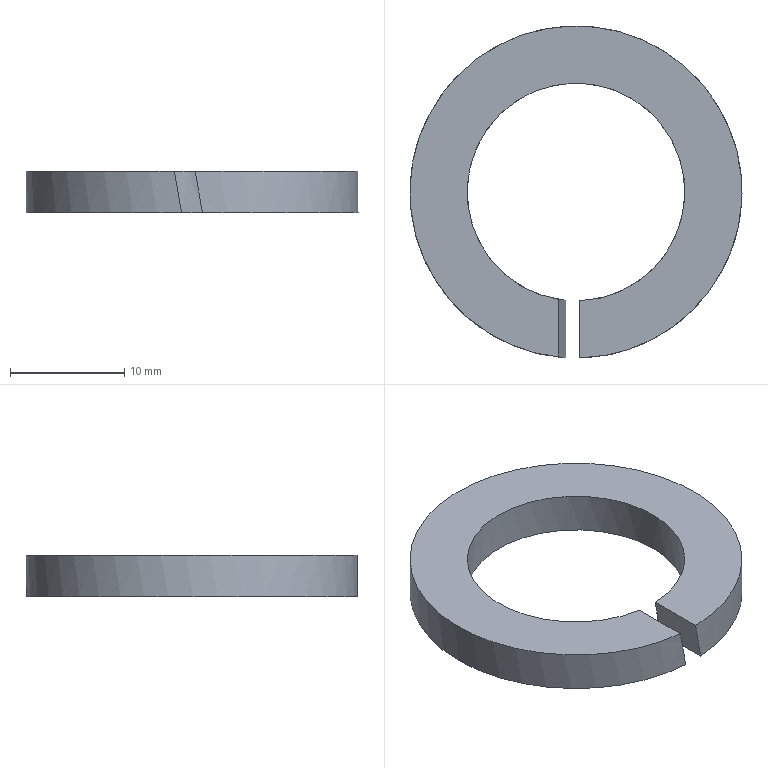Component | NX | GB859-87__18 | 1 solid | 6 faces | box 29.04 x 29.04 x 3.6 mm | volume 1326 mm3 | plane 4 | cylinder 2 | commonest cylinder face diameters 29.04 x1 19.04 x1
STEP:
#1=CARTESIAN_POINT('',(0.,0.,0.));
#2=DIRECTION('',(0.,0.,1.));
#3=DIRECTION('',(1.,0.,0.));
#4=AXIS2_PLACEMENT_3D('',#1,#2,#3);
#5=CARTESIAN_POINT('',(-0.9152,-14.493,110.));
#6=VERTEX_POINT('',#5);
#7=CARTESIAN_POINT('',(0.9125,-14.493,110.));
#8=VERTEX_POINT('',#7);
#9=CARTESIAN_POINT('',(-0.001341,-0.001341,110.));
#10=DIRECTION('',(0.,0.,-1.));
#11=DIRECTION('',(0.,1.,0.));
#12=AXIS2_PLACEMENT_3D('',#9,#10,#11);
#13=CIRCLE('',#12,14.52);
#14=CARTESIAN_POINT('',(-0.001341,-0.001341,110.));
#15=DIRECTION('',(0.,0.,-1.));
#16=DIRECTION('',(0.,1.,0.));
#17=AXIS2_PLACEMENT_3D('',#14,#15,#16);
#18=CYLINDRICAL_SURFACE('',#17,14.52);
#19=CARTESIAN_POINT('',(-6.283,0.));
#20=DIRECTION('',(1.,0.));
#21=VECTOR('',#20,1.);
#22=LINE('',#19,#21);
#23=(GEOMETRIC_REPRESENTATION_CONTEXT(2)PARAMETRIC_REPRESENTATION_CONTEXT()REPRESENTATION_CONTEXT('',''));
#24=DEFINITIONAL_REPRESENTATION('',(#22),#23);
#25=PCURVE('',#18,#24);
#26=CARTESIAN_POINT('',(9.519,-0.001341,110.));
#27=DIRECTION('',(0.,0.,-1.));
#28=DIRECTION('',(0.,1.,0.));
#29=AXIS2_PLACEMENT_3D('',#26,#27,#28);
#30=PLANE('',#29);
#31=CARTESIAN_POINT('',(0.,-9.52));
#32=DIRECTION('',(1.,0.));
#33=AXIS2_PLACEMENT_2D('',#31,#32);
#34=CIRCLE('',#33,14.52);
#35=(GEOMETRIC_REPRESENTATION_CONTEXT(2)PARAMETRIC_REPRESENTATION_CONTEXT()REPRESENTATION_CONTEXT('',''));
#36=DEFINITIONAL_REPRESENTATION('',(#34),#35);
#37=PCURVE('',#30,#36);
#38=SURFACE_CURVE('',#13,(#25,#37),.PCURVE_S1.);
#39=EDGE_CURVE('',#6,#8,#38,.T.);
#40=ORIENTED_EDGE('',*,*,#39,.F.);
#41=CARTESIAN_POINT('',(-1.55,-14.439,113.6));
#42=VERTEX_POINT('',#41);
#43=CARTESIAN_POINT('',(-0.001341,-0.001341,104.817));
#44=DIRECTION('',(-0.9848,0.,-0.1736));
#45=DIRECTION('',(0.1736,0.,-0.9848));
#46=AXIS2_PLACEMENT_3D('',#43,#44,#45);
#47=ELLIPSE('',#46,83.617,14.52);
#48=CARTESIAN_POINT('',(-3.079,-0.));
#49=CARTESIAN_POINT('',(-3.035,-3.6));
#50=B_SPLINE_CURVE_WITH_KNOTS('',1,(#48,#49),.UNSPECIFIED.,.F.,.F.,(2,2),(1.634,1.678),.PIECEWISE_BEZIER_KNOTS.);
#51=(GEOMETRIC_REPRESENTATION_CONTEXT(2)PARAMETRIC_REPRESENTATION_CONTEXT()REPRESENTATION_CONTEXT('',''));
#52=DEFINITIONAL_REPRESENTATION('',(#50),#51);
#53=PCURVE('',#18,#52);
#54=CARTESIAN_POINT('',(-2.19,-21.781,117.23));
#55=DIRECTION('',(0.9848,0.,0.1736));
#56=DIRECTION('',(-0.1736,0.,0.9848));
#57=AXIS2_PLACEMENT_3D('',#54,#55,#56);
#58=PLANE('',#57);
#59=CARTESIAN_POINT('',(-96.222,-21.78));
#60=CARTESIAN_POINT('',(-96.222,3.369));
#61=CARTESIAN_POINT('',(29.205,-9.205));
#62=CARTESIAN_POINT('',(154.631,-21.78));
#63=CARTESIAN_POINT('',(29.205,-34.355));
#64=CARTESIAN_POINT('',(-96.222,-46.929));
#65=CARTESIAN_POINT('',(-96.222,-21.78));
#66=(BOUNDED_CURVE()B_SPLINE_CURVE(2,(#59,#60,#61,#62,#63,#64,#65),.UNSPECIFIED.,.T.,.F.)B_SPLINE_CURVE_WITH_KNOTS((1,2,2,2,2,1),(-2.094,0.,2.094,4.189,6.283,8.378),.UNSPECIFIED.)CURVE()GEOMETRIC_REPRESENTATION_ITEM()RATIONAL_B_SPLINE_CURVE((1.,0.5,1.,0.5,1.,0.5,1.))REPRESENTATION_ITEM(''));
#67=(GEOMETRIC_REPRESENTATION_CONTEXT(2)PARAMETRIC_REPRESENTATION_CONTEXT()REPRESENTATION_CONTEXT('',''));
#68=DEFINITIONAL_REPRESENTATION('',(#66),#67);
#69=PCURVE('',#58,#68);
#70=SURFACE_CURVE('',#47,(#53,#69),.PCURVE_S1.);
#71=EDGE_CURVE('',#6,#42,#70,.T.);
#72=ORIENTED_EDGE('',*,*,#71,.T.);
#73=CARTESIAN_POINT('',(0.2778,-14.519,113.6));
#74=VERTEX_POINT('',#73);
#75=CARTESIAN_POINT('',(-0.001341,-0.001341,113.6));
#76=DIRECTION('',(0.,0.,-1.));
#77=DIRECTION('',(0.,1.,0.));
#78=AXIS2_PLACEMENT_3D('',#75,#76,#77);
#79=CIRCLE('',#78,14.52);
#80=CARTESIAN_POINT('',(-6.283,-3.6));
#81=DIRECTION('',(1.,0.));
#82=VECTOR('',#81,1.);
#83=LINE('',#80,#82);
#84=(GEOMETRIC_REPRESENTATION_CONTEXT(2)PARAMETRIC_REPRESENTATION_CONTEXT()REPRESENTATION_CONTEXT('',''));
#85=DEFINITIONAL_REPRESENTATION('',(#83),#84);
#86=PCURVE('',#18,#85);
#87=CARTESIAN_POINT('',(14.519,-0.001341,113.6));
#88=DIRECTION('',(0.,0.,1.));
#89=DIRECTION('',(0.,-1.,0.));
#90=AXIS2_PLACEMENT_3D('',#87,#88,#89);
#91=PLANE('',#90);
#92=CARTESIAN_POINT('',(-14.52,-14.52));
#93=CARTESIAN_POINT('',(-14.52,10.629));
#94=CARTESIAN_POINT('',(7.26,-1.945));
#95=CARTESIAN_POINT('',(29.04,-14.52));
#96=CARTESIAN_POINT('',(7.26,-27.095));
#97=CARTESIAN_POINT('',(-14.52,-39.669));
#98=CARTESIAN_POINT('',(-14.52,-14.52));
#99=(BOUNDED_CURVE()B_SPLINE_CURVE(2,(#92,#93,#94,#95,#96,#97,#98),.UNSPECIFIED.,.T.,.F.)B_SPLINE_CURVE_WITH_KNOTS((1,2,2,2,2,1),(-2.094,0.,2.094,4.189,6.283,8.378),.UNSPECIFIED.)CURVE()GEOMETRIC_REPRESENTATION_ITEM()RATIONAL_B_SPLINE_CURVE((1.,0.5,1.,0.5,1.,0.5,1.))REPRESENTATION_ITEM(''));
#100=(GEOMETRIC_REPRESENTATION_CONTEXT(2)PARAMETRIC_REPRESENTATION_CONTEXT()REPRESENTATION_CONTEXT('',''));
#101=DEFINITIONAL_REPRESENTATION('',(#99),#100);
#102=PCURVE('',#91,#101);
#103=SURFACE_CURVE('',#79,(#86,#102),.PCURVE_S1.);
#104=EDGE_CURVE('',#42,#74,#103,.T.);
#105=ORIENTED_EDGE('',*,*,#104,.T.);
#106=CARTESIAN_POINT('',(-0.001341,-0.001341,115.183));
#107=DIRECTION('',(0.9848,0.,0.1736));
#108=DIRECTION('',(0.1736,0.,-0.9848));
#109=AXIS2_PLACEMENT_3D('',#106,#107,#108);
#110=ELLIPSE('',#109,83.617,14.52);
#111=CARTESIAN_POINT('',(3.122,-3.6));
#112=CARTESIAN_POINT('',(3.079,0.));
#113=B_SPLINE_CURVE_WITH_KNOTS('',1,(#111,#112),.UNSPECIFIED.,.F.,.F.,(2,2),(4.732,4.775),.PIECEWISE_BEZIER_KNOTS.);
#114=(GEOMETRIC_REPRESENTATION_CONTEXT(2)PARAMETRIC_REPRESENTATION_CONTEXT()REPRESENTATION_CONTEXT('',''));
#115=DEFINITIONAL_REPRESENTATION('',(#113),#114);
#116=PCURVE('',#18,#115);
#117=CARTESIAN_POINT('',(2.187,-21.781,102.77));
#118=DIRECTION('',(-0.9848,0.,-0.1736));
#119=DIRECTION('',(0.1736,0.,-0.9848));
#120=AXIS2_PLACEMENT_3D('',#117,#118,#119);
#121=PLANE('',#120);
#122=CARTESIAN_POINT('',(71.013,-21.78));
#123=CARTESIAN_POINT('',(71.013,-46.929));
#124=CARTESIAN_POINT('',(-54.413,-34.355));
#125=CARTESIAN_POINT('',(-179.839,-21.78));
#126=CARTESIAN_POINT('',(-54.413,-9.205));
#127=CARTESIAN_POINT('',(71.013,3.369));
#128=CARTESIAN_POINT('',(71.013,-21.78));
#129=(BOUNDED_CURVE()B_SPLINE_CURVE(2,(#122,#123,#124,#125,#126,#127,#128),.UNSPECIFIED.,.T.,.F.)B_SPLINE_CURVE_WITH_KNOTS((1,2,2,2,2,1),(-2.094,0.,2.094,4.189,6.283,8.378),.UNSPECIFIED.)CURVE()GEOMETRIC_REPRESENTATION_ITEM()RATIONAL_B_SPLINE_CURVE((1.,0.5,1.,0.5,1.,0.5,1.))REPRESENTATION_ITEM(''));
#130=(GEOMETRIC_REPRESENTATION_CONTEXT(2)PARAMETRIC_REPRESENTATION_CONTEXT()REPRESENTATION_CONTEXT('',''));
#131=DEFINITIONAL_REPRESENTATION('',(#129),#130);
#132=PCURVE('',#121,#131);
#133=SURFACE_CURVE('',#110,(#116,#132),.PCURVE_S1.);
#134=EDGE_CURVE('',#74,#8,#133,.T.);
#135=ORIENTED_EDGE('',*,*,#134,.T.);
#136=EDGE_LOOP('',(#40,#72,#105,#135));
#137=FACE_BOUND('',#136,.T.);
#138=ADVANCED_FACE('',(#137),#18,.T.);
#139=ORIENTED_EDGE('',*,*,#104,.F.);
#140=CARTESIAN_POINT('',(-1.55,-9.395,113.6));
#141=VERTEX_POINT('',#140);
#142=CARTESIAN_POINT('',(-1.55,-0.001341,113.6));
#143=DIRECTION('',(0.,1.,0.));
#144=VECTOR('',#143,1.);
#145=LINE('',#142,#144);
#146=CARTESIAN_POINT('',(0.,-16.069));
#147=DIRECTION('',(-1.,0.));
#148=VECTOR('',#147,1.);
#149=LINE('',#146,#148);
#150=(GEOMETRIC_REPRESENTATION_CONTEXT(2)PARAMETRIC_REPRESENTATION_CONTEXT()REPRESENTATION_CONTEXT('',''));
#151=DEFINITIONAL_REPRESENTATION('',(#149),#150);
#152=PCURVE('',#91,#151);
#153=CARTESIAN_POINT('',(-3.686,-21.78));
#154=DIRECTION('',(0.,-1.));
#155=VECTOR('',#154,1.);
#156=LINE('',#153,#155);
#157=(GEOMETRIC_REPRESENTATION_CONTEXT(2)PARAMETRIC_REPRESENTATION_CONTEXT()REPRESENTATION_CONTEXT('',''));
#158=DEFINITIONAL_REPRESENTATION('',(#156),#157);
#159=PCURVE('',#58,#158);
#160=SURFACE_CURVE('',#145,(#152,#159),.PCURVE_S1.);
#161=EDGE_CURVE('',#42,#141,#160,.T.);
#162=ORIENTED_EDGE('',*,*,#161,.T.);
#163=CARTESIAN_POINT('',(0.2778,-9.517,113.6));
#164=VERTEX_POINT('',#163);
#165=CARTESIAN_POINT('',(-0.001341,-0.001341,113.6));
#166=DIRECTION('',(0.,0.,-1.));
#167=DIRECTION('',(0.,1.,0.));
#168=AXIS2_PLACEMENT_3D('',#165,#166,#167);
#169=CIRCLE('',#168,9.52);
#170=CARTESIAN_POINT('',(-9.52,-14.52));
#171=CARTESIAN_POINT('',(-9.52,1.969));
#172=CARTESIAN_POINT('',(4.76,-6.275));
#173=CARTESIAN_POINT('',(19.04,-14.52));
#174=CARTESIAN_POINT('',(4.76,-22.765));
#175=CARTESIAN_POINT('',(-9.52,-31.009));
#176=CARTESIAN_POINT('',(-9.52,-14.52));
#177=(BOUNDED_CURVE()B_SPLINE_CURVE(2,(#170,#171,#172,#173,#174,#175,#176),.UNSPECIFIED.,.T.,.F.)B_SPLINE_CURVE_WITH_KNOTS((1,2,2,2,2,1),(-2.094,0.,2.094,4.189,6.283,8.378),.UNSPECIFIED.)CURVE()GEOMETRIC_REPRESENTATION_ITEM()RATIONAL_B_SPLINE_CURVE((1.,0.5,1.,0.5,1.,0.5,1.))REPRESENTATION_ITEM(''));
#178=(GEOMETRIC_REPRESENTATION_CONTEXT(2)PARAMETRIC_REPRESENTATION_CONTEXT()REPRESENTATION_CONTEXT('',''));
#179=DEFINITIONAL_REPRESENTATION('',(#177),#178);
#180=PCURVE('',#91,#179);
#181=CARTESIAN_POINT('',(-0.001341,-0.001341,110.));
#182=DIRECTION('',(0.,0.,-1.));
#183=DIRECTION('',(0.,1.,0.));
#184=AXIS2_PLACEMENT_3D('',#181,#182,#183);
#185=CYLINDRICAL_SURFACE('',#184,9.52);
#186=CARTESIAN_POINT('',(-6.283,-3.6));
#187=DIRECTION('',(1.,0.));
#188=VECTOR('',#187,1.);
#189=LINE('',#186,#188);
#190=(GEOMETRIC_REPRESENTATION_CONTEXT(2)PARAMETRIC_REPRESENTATION_CONTEXT()REPRESENTATION_CONTEXT('',''));
#191=DEFINITIONAL_REPRESENTATION('',(#189),#190);
#192=PCURVE('',#185,#191);
#193=SURFACE_CURVE('',#169,(#180,#192),.PCURVE_S1.);
#194=EDGE_CURVE('',#141,#164,#193,.T.);
#195=ORIENTED_EDGE('',*,*,#194,.T.);
#196=CARTESIAN_POINT('',(0.2778,-0.001341,113.6));
#197=DIRECTION('',(0.,-1.,0.));
#198=VECTOR('',#197,1.);
#199=LINE('',#196,#198);
#200=CARTESIAN_POINT('',(0.,-14.241));
#201=DIRECTION('',(1.,0.));
#202=VECTOR('',#201,1.);
#203=LINE('',#200,#202);
#204=(GEOMETRIC_REPRESENTATION_CONTEXT(2)PARAMETRIC_REPRESENTATION_CONTEXT()REPRESENTATION_CONTEXT('',''));
#205=DEFINITIONAL_REPRESENTATION('',(#203),#204);
#206=PCURVE('',#91,#205);
#207=CARTESIAN_POINT('',(-10.997,-21.78));
#208=DIRECTION('',(0.,1.));
#209=VECTOR('',#208,1.);
#210=LINE('',#207,#209);
#211=(GEOMETRIC_REPRESENTATION_CONTEXT(2)PARAMETRIC_REPRESENTATION_CONTEXT()REPRESENTATION_CONTEXT('',''));
#212=DEFINITIONAL_REPRESENTATION('',(#210),#211);
#213=PCURVE('',#121,#212);
#214=SURFACE_CURVE('',#199,(#206,#213),.PCURVE_S1.);
#215=EDGE_CURVE('',#164,#74,#214,.T.);
#216=ORIENTED_EDGE('',*,*,#215,.T.);
#217=EDGE_LOOP('',(#139,#162,#195,#216));
#218=FACE_BOUND('',#217,.T.);
#219=ADVANCED_FACE('',(#218),#91,.T.);
#220=CARTESIAN_POINT('',(0.9125,-9.477,110.));
#221=VERTEX_POINT('',#220);
#222=CARTESIAN_POINT('',(-0.001341,-0.001341,115.183));
#223=DIRECTION('',(-0.9848,0.,-0.1736));
#224=DIRECTION('',(0.1736,0.,-0.9848));
#225=AXIS2_PLACEMENT_3D('',#222,#223,#224);
#226=ELLIPSE('',#225,54.823,9.52);
#227=CARTESIAN_POINT('',(3.045,0.));
#228=CARTESIAN_POINT('',(3.112,-3.6));
#229=B_SPLINE_CURVE_WITH_KNOTS('',1,(#227,#228),.UNSPECIFIED.,.F.,.F.,(2,2),(1.475,1.541),.PIECEWISE_BEZIER_KNOTS.);
#230=(GEOMETRIC_REPRESENTATION_CONTEXT(2)PARAMETRIC_REPRESENTATION_CONTEXT()REPRESENTATION_CONTEXT('',''));
#231=DEFINITIONAL_REPRESENTATION('',(#229),#230);
#232=PCURVE('',#185,#231);
#233=CARTESIAN_POINT('',(-12.604,-21.78));
#234=DIRECTION('',(1.,0.));
#235=AXIS2_PLACEMENT_2D('',#233,#234);
#236=ELLIPSE('',#235,54.823,9.52);
#237=(GEOMETRIC_REPRESENTATION_CONTEXT(2)PARAMETRIC_REPRESENTATION_CONTEXT()REPRESENTATION_CONTEXT('',''));
#238=DEFINITIONAL_REPRESENTATION('',(#236),#237);
#239=PCURVE('',#121,#238);
#240=SURFACE_CURVE('',#226,(#232,#239),.PCURVE_S1.);
#241=EDGE_CURVE('',#221,#164,#240,.T.);
#242=ORIENTED_EDGE('',*,*,#241,.F.);
#243=CARTESIAN_POINT('',(-0.9152,-9.477,110.));
#244=VERTEX_POINT('',#243);
#245=CARTESIAN_POINT('',(-0.001341,-0.001341,110.));
#246=DIRECTION('',(0.,0.,-1.));
#247=DIRECTION('',(0.,1.,0.));
#248=AXIS2_PLACEMENT_3D('',#245,#246,#247);
#249=CIRCLE('',#248,9.52);
#250=CARTESIAN_POINT('',(-6.283,0.));
#251=DIRECTION('',(1.,0.));
#252=VECTOR('',#251,1.);
#253=LINE('',#250,#252);
#254=(GEOMETRIC_REPRESENTATION_CONTEXT(2)PARAMETRIC_REPRESENTATION_CONTEXT()REPRESENTATION_CONTEXT('',''));
#255=DEFINITIONAL_REPRESENTATION('',(#253),#254);
#256=PCURVE('',#185,#255);
#257=CARTESIAN_POINT('',(0.,-9.52));
#258=DIRECTION('',(1.,0.));
#259=AXIS2_PLACEMENT_2D('',#257,#258);
#260=CIRCLE('',#259,9.52);
#261=(GEOMETRIC_REPRESENTATION_CONTEXT(2)PARAMETRIC_REPRESENTATION_CONTEXT()REPRESENTATION_CONTEXT('',''));
#262=DEFINITIONAL_REPRESENTATION('',(#260),#261);
#263=PCURVE('',#30,#262);
#264=SURFACE_CURVE('',#249,(#256,#263),.PCURVE_S1.);
#265=EDGE_CURVE('',#244,#221,#264,.T.);
#266=ORIENTED_EDGE('',*,*,#265,.F.);
#267=CARTESIAN_POINT('',(-0.001341,-0.001341,104.817));
#268=DIRECTION('',(0.9848,0.,0.1736));
#269=DIRECTION('',(0.1736,0.,-0.9848));
#270=AXIS2_PLACEMENT_3D('',#267,#268,#269);
#271=ELLIPSE('',#270,54.823,9.52);
#272=CARTESIAN_POINT('',(-2.978,-3.6));
#273=CARTESIAN_POINT('',(-3.045,0.));
#274=B_SPLINE_CURVE_WITH_KNOTS('',1,(#272,#273),.UNSPECIFIED.,.F.,.F.,(2,2),(4.549,4.616),.PIECEWISE_BEZIER_KNOTS.);
#275=(GEOMETRIC_REPRESENTATION_CONTEXT(2)PARAMETRIC_REPRESENTATION_CONTEXT()REPRESENTATION_CONTEXT('',''));
#276=DEFINITIONAL_REPRESENTATION('',(#274),#275);
#277=PCURVE('',#185,#276);
#278=CARTESIAN_POINT('',(-12.604,-21.78));
#279=DIRECTION('',(-1.,0.));
#280=AXIS2_PLACEMENT_2D('',#278,#279);
#281=ELLIPSE('',#280,54.823,9.52);
#282=(GEOMETRIC_REPRESENTATION_CONTEXT(2)PARAMETRIC_REPRESENTATION_CONTEXT()REPRESENTATION_CONTEXT('',''));
#283=DEFINITIONAL_REPRESENTATION('',(#281),#282);
#284=PCURVE('',#58,#283);
#285=SURFACE_CURVE('',#271,(#277,#284),.PCURVE_S1.);
#286=EDGE_CURVE('',#141,#244,#285,.T.);
#287=ORIENTED_EDGE('',*,*,#286,.F.);
#288=ORIENTED_EDGE('',*,*,#194,.T.);
#289=EDGE_LOOP('',(#242,#266,#287,#288));
#290=FACE_BOUND('',#289,.F.);
#291=ADVANCED_FACE('',(#290),#185,.F.);
#292=ORIENTED_EDGE('',*,*,#265,.F.);
#293=CARTESIAN_POINT('',(-0.9152,-0.001341,110.));
#294=DIRECTION('',(0.,-1.,0.));
#295=VECTOR('',#294,1.);
#296=LINE('',#293,#295);
#297=CARTESIAN_POINT('',(0.,-10.434));
#298=DIRECTION('',(-1.,0.));
#299=VECTOR('',#298,1.);
#300=LINE('',#297,#299);
#301=(GEOMETRIC_REPRESENTATION_CONTEXT(2)PARAMETRIC_REPRESENTATION_CONTEXT()REPRESENTATION_CONTEXT('',''));
#302=DEFINITIONAL_REPRESENTATION('',(#300),#301);
#303=PCURVE('',#30,#302);
#304=CARTESIAN_POINT('',(-7.341,-21.78));
#305=DIRECTION('',(0.,1.));
#306=VECTOR('',#305,1.);
#307=LINE('',#304,#306);
#308=(GEOMETRIC_REPRESENTATION_CONTEXT(2)PARAMETRIC_REPRESENTATION_CONTEXT()REPRESENTATION_CONTEXT('',''));
#309=DEFINITIONAL_REPRESENTATION('',(#307),#308);
#310=PCURVE('',#58,#309);
#311=SURFACE_CURVE('',#296,(#303,#310),.PCURVE_S1.);
#312=EDGE_CURVE('',#244,#6,#311,.T.);
#313=ORIENTED_EDGE('',*,*,#312,.T.);
#314=ORIENTED_EDGE('',*,*,#39,.T.);
#315=CARTESIAN_POINT('',(0.9125,-0.001341,110.));
#316=DIRECTION('',(0.,1.,0.));
#317=VECTOR('',#316,1.);
#318=LINE('',#315,#317);
#319=CARTESIAN_POINT('',(0.,-8.606));
#320=DIRECTION('',(1.,0.));
#321=VECTOR('',#320,1.);
#322=LINE('',#319,#321);
#323=(GEOMETRIC_REPRESENTATION_CONTEXT(2)PARAMETRIC_REPRESENTATION_CONTEXT()REPRESENTATION_CONTEXT('',''));
#324=DEFINITIONAL_REPRESENTATION('',(#322),#323);
#325=PCURVE('',#30,#324);
#326=CARTESIAN_POINT('',(-7.341,-21.78));
#327=DIRECTION('',(0.,-1.));
#328=VECTOR('',#327,1.);
#329=LINE('',#326,#328);
#330=(GEOMETRIC_REPRESENTATION_CONTEXT(2)PARAMETRIC_REPRESENTATION_CONTEXT()REPRESENTATION_CONTEXT('',''));
#331=DEFINITIONAL_REPRESENTATION('',(#329),#330);
#332=PCURVE('',#121,#331);
#333=SURFACE_CURVE('',#318,(#325,#332),.PCURVE_S1.);
#334=EDGE_CURVE('',#8,#221,#333,.T.);
#335=ORIENTED_EDGE('',*,*,#334,.T.);
#336=EDGE_LOOP('',(#292,#313,#314,#335));
#337=FACE_BOUND('',#336,.T.);
#338=ADVANCED_FACE('',(#337),#30,.T.);
#339=ORIENTED_EDGE('',*,*,#215,.F.);
#340=ORIENTED_EDGE('',*,*,#241,.F.);
#341=ORIENTED_EDGE('',*,*,#334,.F.);
#342=ORIENTED_EDGE('',*,*,#134,.F.);
#343=EDGE_LOOP('',(#339,#340,#341,#342));
#344=FACE_BOUND('',#343,.T.);
#345=ADVANCED_FACE('',(#344),#121,.T.);
#346=ORIENTED_EDGE('',*,*,#312,.F.);
#347=ORIENTED_EDGE('',*,*,#286,.F.);
#348=ORIENTED_EDGE('',*,*,#161,.F.);
#349=ORIENTED_EDGE('',*,*,#71,.F.);
#350=EDGE_LOOP('',(#346,#347,#348,#349));
#351=FACE_BOUND('',#350,.T.);
#352=ADVANCED_FACE('',(#351),#58,.T.);
#353=CLOSED_SHELL('',(#138,#219,#291,#338,#345,#352));
#354=MANIFOLD_SOLID_BREP('',#353);
#355=(LENGTH_UNIT()NAMED_UNIT(*)SI_UNIT(.MILLI.,.METRE.));
#356=UNCERTAINTY_MEASURE_WITH_UNIT(LENGTH_MEASURE(0.002),#355,'','');
#357=(NAMED_UNIT(*)PLANE_ANGLE_UNIT()SI_UNIT($,.RADIAN.));
#358=(NAMED_UNIT(*)SI_UNIT($,.STERADIAN.)SOLID_ANGLE_UNIT());
#359=(GEOMETRIC_REPRESENTATION_CONTEXT(3)GLOBAL_UNCERTAINTY_ASSIGNED_CONTEXT((#356))GLOBAL_UNIT_ASSIGNED_CONTEXT((#355,#357,#358))REPRESENTATION_CONTEXT('',''));
#360=ADVANCED_BREP_SHAPE_REPRESENTATION('',(#4,#354),#359);